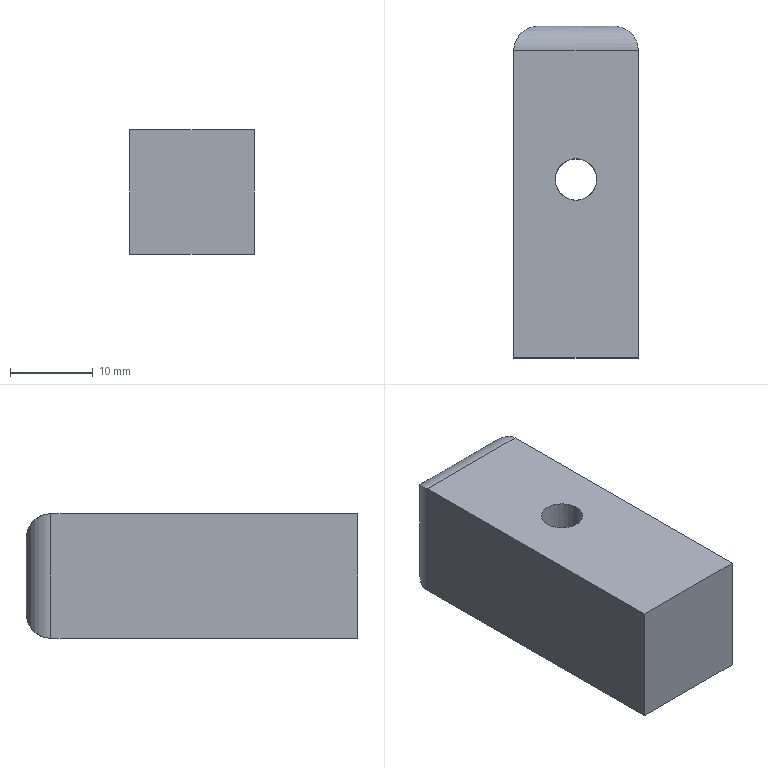Component | SolidWorks | SlideRailSupport-1 | 1 solid | 19 faces | box 15 x 40 x 15 mm | volume 8467 mm3 | cylinder 12 | plane 7 | commonest cylinder face diameters 5 x8 6 x4
build123d program:
from build123d import *

# Parameters (mm, degrees)
SKETCH1_W           = 15
SKETCH1_H           = 15
BOSS_EXTRUDE1_DEPTH = 20
FILLET1_R           = 3
SKETCH2_R           = 2.5
CUT_EXTRUDE1_DEPTH  = 25
SKETCH3_R           = 2.5
CUT_EXTRUDE2_DEPTH  = 11


with BuildPart() as part:
    # Sketch1 → Boss-Extrude1 (new, symmetric)
    with BuildSketch(Plane(origin=(0, 0, 0), x_dir=(0, 0, -1), z_dir=(1, 0, 0))):
        Rectangle(SKETCH1_W, SKETCH1_H)
    extrude(amount=BOSS_EXTRUDE1_DEPTH, both=True)

    # Fillet1
    fillet1_edges = [part.edges().sort_by_distance(p)[0] for p in [
        (-20, -7.5, 0),
        (-20, 0, 7.5),
        (-20, 7.5, 0),
        (-20, 0, -7.5),
    ]]
    fillet(fillet1_edges, radius=FILLET1_R)

    # Sketch2 → Cut-Extrude1 (cut, symmetric)
    with BuildSketch(Plane(origin=(0, 7.5, 0), x_dir=(1, 0, 0), z_dir=(0, 1, 0))):
        with Locations(Location((-1.5, 0, 0), (0, 0, 270))):
            Circle(SKETCH2_R)
    extrude(amount=CUT_EXTRUDE1_DEPTH, both=True, mode=Mode.SUBTRACT)

    # Sketch3 → Cut-Extrude2 (cut)
    with BuildSketch(Plane(origin=(0, 0, -7.5), x_dir=(-1, 0, 0), z_dir=(0, 0, -1))):
        with Locations(Location((1.5, 0, 0), (0, 0, 90))):
            Circle(SKETCH3_R)
    extrude(amount=-CUT_EXTRUDE2_DEPTH, mode=Mode.SUBTRACT)


solid = part.part

# Placed as in the assembly
solid = solid.moved(Location((-191.5, 218.5, 125), (90, -90, 0)))
STEP:
#1=CARTESIAN_POINT('',(-7.677,8.661,4.823));
#2=VERTEX_POINT('',#1);
#3=CARTESIAN_POINT('',(-7.677,8.661,5.02));
#4=VERTEX_POINT('',#3);
#5=CARTESIAN_POINT('',(-7.677,8.661,4.921));
#6=DIRECTION('',(1.,0.,0.));
#7=DIRECTION('',(0.,0.,1.));
#8=AXIS2_PLACEMENT_3D('',#5,#6,#7);
#9=CIRCLE('',#8,0.09843);
#10=EDGE_CURVE('',#2,#4,#9,.T.);
#11=ORIENTED_EDGE('',*,*,#10,.F.);
#12=CARTESIAN_POINT('',(-7.638,8.661,4.823));
#13=VERTEX_POINT('',#12);
#14=CARTESIAN_POINT('',(-7.677,8.661,4.823));
#15=DIRECTION('',(1.,0.,0.));
#16=VECTOR('',#15,39.37);
#17=LINE('',#14,#16);
#18=EDGE_CURVE('',#2,#13,#17,.T.);
#19=ORIENTED_EDGE('',*,*,#18,.T.);
#20=CARTESIAN_POINT('',(-7.539,8.76,4.921));
#21=VERTEX_POINT('',#20);
#22=CARTESIAN_POINT('',(-7.539,8.76,4.921));
#23=CARTESIAN_POINT('',(-7.597,8.76,4.864));
#24=CARTESIAN_POINT('',(-7.638,8.719,4.823));
#25=CARTESIAN_POINT('',(-7.638,8.661,4.823));
#26=(BOUNDED_CURVE()B_SPLINE_CURVE(3,(#22,#23,#24,#25),.UNSPECIFIED.,.F.,.T.)B_SPLINE_CURVE_WITH_KNOTS((4,4),(1.571,3.142),.UNSPECIFIED.)CURVE()GEOMETRIC_REPRESENTATION_ITEM()RATIONAL_B_SPLINE_CURVE((1.,0.8047,0.8047,1.))REPRESENTATION_ITEM(''));
#27=EDGE_CURVE('',#21,#13,#26,.T.);
#28=ORIENTED_EDGE('',*,*,#27,.F.);
#29=CARTESIAN_POINT('',(-7.638,8.661,5.02));
#30=VERTEX_POINT('',#29);
#31=CARTESIAN_POINT('',(-7.638,8.661,5.02));
#32=CARTESIAN_POINT('',(-7.638,8.719,5.02));
#33=CARTESIAN_POINT('',(-7.597,8.76,4.979));
#34=CARTESIAN_POINT('',(-7.539,8.76,4.921));
#35=(BOUNDED_CURVE()B_SPLINE_CURVE(3,(#31,#32,#33,#34),.UNSPECIFIED.,.F.,.T.)B_SPLINE_CURVE_WITH_KNOTS((4,4),(0.,1.571),.UNSPECIFIED.)CURVE()GEOMETRIC_REPRESENTATION_ITEM()RATIONAL_B_SPLINE_CURVE((1.,0.8047,0.8047,1.))REPRESENTATION_ITEM(''));
#36=EDGE_CURVE('',#30,#21,#35,.T.);
#37=ORIENTED_EDGE('',*,*,#36,.F.);
#38=CARTESIAN_POINT('',(-7.677,8.661,5.02));
#39=DIRECTION('',(1.,0.,0.));
#40=VECTOR('',#39,39.37);
#41=LINE('',#38,#40);
#42=EDGE_CURVE('',#4,#30,#41,.T.);
#43=ORIENTED_EDGE('',*,*,#42,.F.);
#44=EDGE_LOOP('',(#11,#19,#28,#37,#43));
#45=FACE_OUTER_BOUND('',#44,.T.);
#46=CARTESIAN_POINT('',(-7.677,8.661,4.921));
#47=DIRECTION('',(1.,0.,0.));
#48=DIRECTION('',(0.,0.,1.));
#49=AXIS2_PLACEMENT_3D('',#46,#47,#48);
#50=CYLINDRICAL_SURFACE('',#49,0.09843);
#51=ADVANCED_FACE('',(#45),#50,.F.);
#52=CARTESIAN_POINT('',(-7.441,8.661,4.823));
#53=VERTEX_POINT('',#52);
#54=CARTESIAN_POINT('',(-7.441,8.661,4.823));
#55=CARTESIAN_POINT('',(-7.441,8.719,4.823));
#56=CARTESIAN_POINT('',(-7.482,8.76,4.864));
#57=CARTESIAN_POINT('',(-7.539,8.76,4.921));
#58=(BOUNDED_CURVE()B_SPLINE_CURVE(3,(#54,#55,#56,#57),.UNSPECIFIED.,.F.,.F.)B_SPLINE_CURVE_WITH_KNOTS((4,4),(3.142,4.712),.UNSPECIFIED.)CURVE()GEOMETRIC_REPRESENTATION_ITEM()RATIONAL_B_SPLINE_CURVE((1.,0.8047,0.8047,1.))REPRESENTATION_ITEM(''));
#59=EDGE_CURVE('',#53,#21,#58,.T.);
#60=ORIENTED_EDGE('',*,*,#59,.F.);
#61=CARTESIAN_POINT('',(-7.244,8.661,4.823));
#62=VERTEX_POINT('',#61);
#63=CARTESIAN_POINT('',(-7.677,8.661,4.823));
#64=DIRECTION('',(1.,0.,0.));
#65=VECTOR('',#64,39.37);
#66=LINE('',#63,#65);
#67=EDGE_CURVE('',#53,#62,#66,.T.);
#68=ORIENTED_EDGE('',*,*,#67,.T.);
#69=CARTESIAN_POINT('',(-7.244,8.661,5.02));
#70=VERTEX_POINT('',#69);
#71=CARTESIAN_POINT('',(-7.244,8.661,4.921));
#72=DIRECTION('',(1.,0.,0.));
#73=DIRECTION('',(0.,0.,1.));
#74=AXIS2_PLACEMENT_3D('',#71,#72,#73);
#75=CIRCLE('',#74,0.09843);
#76=EDGE_CURVE('',#62,#70,#75,.T.);
#77=ORIENTED_EDGE('',*,*,#76,.T.);
#78=CARTESIAN_POINT('',(-7.441,8.661,5.02));
#79=VERTEX_POINT('',#78);
#80=CARTESIAN_POINT('',(-7.677,8.661,5.02));
#81=DIRECTION('',(1.,0.,0.));
#82=VECTOR('',#81,39.37);
#83=LINE('',#80,#82);
#84=EDGE_CURVE('',#79,#70,#83,.T.);
#85=ORIENTED_EDGE('',*,*,#84,.F.);
#86=CARTESIAN_POINT('',(-7.539,8.76,4.921));
#87=CARTESIAN_POINT('',(-7.482,8.76,4.979));
#88=CARTESIAN_POINT('',(-7.441,8.719,5.02));
#89=CARTESIAN_POINT('',(-7.441,8.661,5.02));
#90=(BOUNDED_CURVE()B_SPLINE_CURVE(3,(#86,#87,#88,#89),.UNSPECIFIED.,.F.,.F.)B_SPLINE_CURVE_WITH_KNOTS((4,4),(4.712,6.283),.UNSPECIFIED.)CURVE()GEOMETRIC_REPRESENTATION_ITEM()RATIONAL_B_SPLINE_CURVE((1.,0.8047,0.8047,1.))REPRESENTATION_ITEM(''));
#91=EDGE_CURVE('',#21,#79,#90,.T.);
#92=ORIENTED_EDGE('',*,*,#91,.F.);
#93=EDGE_LOOP('',(#60,#68,#77,#85,#92));
#94=FACE_OUTER_BOUND('',#93,.T.);
#95=CARTESIAN_POINT('',(-7.677,8.661,4.921));
#96=DIRECTION('',(1.,0.,0.));
#97=DIRECTION('',(0.,0.,1.));
#98=AXIS2_PLACEMENT_3D('',#95,#96,#97);
#99=CYLINDRICAL_SURFACE('',#98,0.09843);
#100=ADVANCED_FACE('',(#94),#99,.F.);
#101=CARTESIAN_POINT('',(-7.441,8.661,4.626));
#102=VERTEX_POINT('',#101);
#103=CARTESIAN_POINT('',(-7.638,8.661,4.626));
#104=VERTEX_POINT('',#103);
#105=CARTESIAN_POINT('',(-7.539,8.661,4.626));
#106=DIRECTION('',(0.,0.,1.));
#107=DIRECTION('',(-1.,0.,0.));
#108=AXIS2_PLACEMENT_3D('',#105,#106,#107);
#109=CIRCLE('',#108,0.09843);
#110=EDGE_CURVE('',#102,#104,#109,.T.);
#111=ORIENTED_EDGE('',*,*,#110,.F.);
#112=CARTESIAN_POINT('',(-7.441,8.661,4.232));
#113=DIRECTION('',(-0.,0.,1.));
#114=VECTOR('',#113,39.37);
#115=LINE('',#112,#114);
#116=EDGE_CURVE('',#102,#53,#115,.T.);
#117=ORIENTED_EDGE('',*,*,#116,.T.);
#118=ORIENTED_EDGE('',*,*,#59,.T.);
#119=ORIENTED_EDGE('',*,*,#27,.T.);
#120=CARTESIAN_POINT('',(-7.638,8.661,4.232));
#121=DIRECTION('',(-0.,0.,1.));
#122=VECTOR('',#121,39.37);
#123=LINE('',#120,#122);
#124=EDGE_CURVE('',#104,#13,#123,.T.);
#125=ORIENTED_EDGE('',*,*,#124,.F.);
#126=EDGE_LOOP('',(#111,#117,#118,#119,#125));
#127=FACE_OUTER_BOUND('',#126,.T.);
#128=CARTESIAN_POINT('',(-7.539,8.661,4.232));
#129=DIRECTION('',(-0.,0.,1.));
#130=DIRECTION('',(-1.,0.,0.));
#131=AXIS2_PLACEMENT_3D('',#128,#129,#130);
#132=CYLINDRICAL_SURFACE('',#131,0.09843);
#133=ADVANCED_FACE('',(#127),#132,.F.);
#134=ORIENTED_EDGE('',*,*,#91,.T.);
#135=CARTESIAN_POINT('',(-7.441,8.661,5.217));
#136=VERTEX_POINT('',#135);
#137=CARTESIAN_POINT('',(-7.441,8.661,4.232));
#138=DIRECTION('',(-0.,0.,1.));
#139=VECTOR('',#138,39.37);
#140=LINE('',#137,#139);
#141=EDGE_CURVE('',#79,#136,#140,.T.);
#142=ORIENTED_EDGE('',*,*,#141,.T.);
#143=CARTESIAN_POINT('',(-7.638,8.661,5.217));
#144=VERTEX_POINT('',#143);
#145=CARTESIAN_POINT('',(-7.539,8.661,5.217));
#146=DIRECTION('',(0.,-0.,-1.));
#147=DIRECTION('',(1.,0.,0.));
#148=AXIS2_PLACEMENT_3D('',#145,#146,#147);
#149=CIRCLE('',#148,0.09843);
#150=EDGE_CURVE('',#144,#136,#149,.T.);
#151=ORIENTED_EDGE('',*,*,#150,.F.);
#152=CARTESIAN_POINT('',(-7.638,8.661,4.232));
#153=DIRECTION('',(-0.,0.,1.));
#154=VECTOR('',#153,39.37);
#155=LINE('',#152,#154);
#156=EDGE_CURVE('',#30,#144,#155,.T.);
#157=ORIENTED_EDGE('',*,*,#156,.F.);
#158=ORIENTED_EDGE('',*,*,#36,.T.);
#159=EDGE_LOOP('',(#134,#142,#151,#157,#158));
#160=FACE_OUTER_BOUND('',#159,.T.);
#161=CARTESIAN_POINT('',(-7.539,8.661,4.232));
#162=DIRECTION('',(-0.,0.,1.));
#163=DIRECTION('',(-1.,0.,0.));
#164=AXIS2_PLACEMENT_3D('',#161,#162,#163);
#165=CYLINDRICAL_SURFACE('',#164,0.09843);
#166=ADVANCED_FACE('',(#160),#165,.F.);
#167=ORIENTED_EDGE('',*,*,#141,.F.);
#168=CARTESIAN_POINT('',(-7.539,8.563,4.921));
#169=VERTEX_POINT('',#168);
#170=CARTESIAN_POINT('',(-7.441,8.661,5.02));
#171=CARTESIAN_POINT('',(-7.441,8.604,5.02));
#172=CARTESIAN_POINT('',(-7.482,8.563,4.979));
#173=CARTESIAN_POINT('',(-7.539,8.563,4.921));
#174=(BOUNDED_CURVE()B_SPLINE_CURVE(3,(#170,#171,#172,#173),.UNSPECIFIED.,.F.,.F.)B_SPLINE_CURVE_WITH_KNOTS((4,4),(0.,1.571),.UNSPECIFIED.)CURVE()GEOMETRIC_REPRESENTATION_ITEM()RATIONAL_B_SPLINE_CURVE((1.,0.8047,0.8047,1.))REPRESENTATION_ITEM(''));
#175=EDGE_CURVE('',#79,#169,#174,.T.);
#176=ORIENTED_EDGE('',*,*,#175,.T.);
#177=CARTESIAN_POINT('',(-7.539,8.563,4.921));
#178=CARTESIAN_POINT('',(-7.597,8.563,4.979));
#179=CARTESIAN_POINT('',(-7.638,8.604,5.02));
#180=CARTESIAN_POINT('',(-7.638,8.661,5.02));
#181=(BOUNDED_CURVE()B_SPLINE_CURVE(3,(#177,#178,#179,#180),.UNSPECIFIED.,.F.,.T.)B_SPLINE_CURVE_WITH_KNOTS((4,4),(4.712,6.283),.UNSPECIFIED.)CURVE()GEOMETRIC_REPRESENTATION_ITEM()RATIONAL_B_SPLINE_CURVE((1.,0.8047,0.8047,1.))REPRESENTATION_ITEM(''));
#182=EDGE_CURVE('',#169,#30,#181,.T.);
#183=ORIENTED_EDGE('',*,*,#182,.T.);
#184=ORIENTED_EDGE('',*,*,#156,.T.);
#185=CARTESIAN_POINT('',(-7.539,8.661,5.217));
#186=DIRECTION('',(0.,-0.,-1.));
#187=DIRECTION('',(1.,0.,0.));
#188=AXIS2_PLACEMENT_3D('',#185,#186,#187);
#189=CIRCLE('',#188,0.09843);
#190=EDGE_CURVE('',#136,#144,#189,.T.);
#191=ORIENTED_EDGE('',*,*,#190,.F.);
#192=EDGE_LOOP('',(#167,#176,#183,#184,#191));
#193=FACE_OUTER_BOUND('',#192,.T.);
#194=CARTESIAN_POINT('',(-7.539,8.661,4.232));
#195=DIRECTION('',(-0.,0.,1.));
#196=DIRECTION('',(-1.,0.,0.));
#197=AXIS2_PLACEMENT_3D('',#194,#195,#196);
#198=CYLINDRICAL_SURFACE('',#197,0.09843);
#199=ADVANCED_FACE('',(#193),#198,.F.);
#200=CARTESIAN_POINT('',(-7.244,8.661,4.921));
#201=DIRECTION('',(1.,0.,0.));
#202=DIRECTION('',(0.,0.,1.));
#203=AXIS2_PLACEMENT_3D('',#200,#201,#202);
#204=CIRCLE('',#203,0.09843);
#205=EDGE_CURVE('',#70,#62,#204,.T.);
#206=ORIENTED_EDGE('',*,*,#205,.F.);
#207=ORIENTED_EDGE('',*,*,#76,.F.);
#208=EDGE_LOOP('',(#206,#207));
#209=FACE_BOUND('',#208,.T.);
#210=CARTESIAN_POINT('',(-7.244,7.815,4.626));
#211=VERTEX_POINT('',#210);
#212=CARTESIAN_POINT('',(-7.244,9.272,4.626));
#213=VERTEX_POINT('',#212);
#214=CARTESIAN_POINT('',(-7.244,7.815,4.626));
#215=DIRECTION('',(-0.,1.,-0.));
#216=VECTOR('',#215,39.37);
#217=LINE('',#214,#216);
#218=EDGE_CURVE('',#211,#213,#217,.T.);
#219=ORIENTED_EDGE('',*,*,#218,.T.);
#220=CARTESIAN_POINT('',(-7.244,9.272,5.217));
#221=VERTEX_POINT('',#220);
#222=CARTESIAN_POINT('',(-7.244,9.272,5.217));
#223=DIRECTION('',(-0.,0.,1.));
#224=VECTOR('',#223,39.37);
#225=LINE('',#222,#224);
#226=EDGE_CURVE('',#213,#221,#225,.T.);
#227=ORIENTED_EDGE('',*,*,#226,.T.);
#228=CARTESIAN_POINT('',(-7.244,7.815,5.217));
#229=VERTEX_POINT('',#228);
#230=CARTESIAN_POINT('',(-7.244,7.815,5.217));
#231=DIRECTION('',(-0.,1.,-0.));
#232=VECTOR('',#231,39.37);
#233=LINE('',#230,#232);
#234=EDGE_CURVE('',#229,#221,#233,.T.);
#235=ORIENTED_EDGE('',*,*,#234,.F.);
#236=CARTESIAN_POINT('',(-7.244,7.815,5.217));
#237=DIRECTION('',(-0.,0.,1.));
#238=VECTOR('',#237,39.37);
#239=LINE('',#236,#238);
#240=EDGE_CURVE('',#211,#229,#239,.T.);
#241=ORIENTED_EDGE('',*,*,#240,.F.);
#242=EDGE_LOOP('',(#219,#227,#235,#241));
#243=FACE_OUTER_BOUND('',#242,.T.);
#244=CARTESIAN_POINT('',(-7.244,7.815,5.217));
#245=DIRECTION('',(-1.,-0.,-0.));
#246=DIRECTION('',(0.,-0.,-1.));
#247=AXIS2_PLACEMENT_3D('',#244,#245,#246);
#248=PLANE('',#247);
#249=ADVANCED_FACE('',(#209,#243),#248,.F.);
#250=ORIENTED_EDGE('',*,*,#150,.T.);
#251=ORIENTED_EDGE('',*,*,#190,.T.);
#252=EDGE_LOOP('',(#250,#251));
#253=FACE_BOUND('',#252,.T.);
#254=ORIENTED_EDGE('',*,*,#234,.T.);
#255=CARTESIAN_POINT('',(-7.835,9.272,5.217));
#256=VERTEX_POINT('',#255);
#257=CARTESIAN_POINT('',(-7.835,9.272,5.217));
#258=DIRECTION('',(-1.,-0.,0.));
#259=VECTOR('',#258,39.37);
#260=LINE('',#257,#259);
#261=EDGE_CURVE('',#221,#256,#260,.T.);
#262=ORIENTED_EDGE('',*,*,#261,.T.);
#263=CARTESIAN_POINT('',(-7.835,7.815,5.217));
#264=VERTEX_POINT('',#263);
#265=CARTESIAN_POINT('',(-7.835,7.815,5.217));
#266=DIRECTION('',(-0.,1.,-0.));
#267=VECTOR('',#266,39.37);
#268=LINE('',#265,#267);
#269=EDGE_CURVE('',#264,#256,#268,.T.);
#270=ORIENTED_EDGE('',*,*,#269,.F.);
#271=CARTESIAN_POINT('',(-7.835,7.815,5.217));
#272=DIRECTION('',(-1.,-0.,0.));
#273=VECTOR('',#272,39.37);
#274=LINE('',#271,#273);
#275=EDGE_CURVE('',#229,#264,#274,.T.);
#276=ORIENTED_EDGE('',*,*,#275,.F.);
#277=EDGE_LOOP('',(#254,#262,#270,#276));
#278=FACE_OUTER_BOUND('',#277,.T.);
#279=CARTESIAN_POINT('',(-7.835,7.815,5.217));
#280=DIRECTION('',(0.,-0.,-1.));
#281=DIRECTION('',(1.,0.,-0.));
#282=AXIS2_PLACEMENT_3D('',#279,#280,#281);
#283=PLANE('',#282);
#284=ADVANCED_FACE('',(#253,#278),#283,.F.);
#285=ORIENTED_EDGE('',*,*,#269,.T.);
#286=CARTESIAN_POINT('',(-7.835,9.272,4.626));
#287=VERTEX_POINT('',#286);
#288=CARTESIAN_POINT('',(-7.835,9.272,5.217));
#289=DIRECTION('',(0.,-0.,-1.));
#290=VECTOR('',#289,39.37);
#291=LINE('',#288,#290);
#292=EDGE_CURVE('',#256,#287,#291,.T.);
#293=ORIENTED_EDGE('',*,*,#292,.T.);
#294=CARTESIAN_POINT('',(-7.835,7.815,4.626));
#295=VERTEX_POINT('',#294);
#296=CARTESIAN_POINT('',(-7.835,7.815,4.626));
#297=DIRECTION('',(-0.,1.,-0.));
#298=VECTOR('',#297,39.37);
#299=LINE('',#296,#298);
#300=EDGE_CURVE('',#295,#287,#299,.T.);
#301=ORIENTED_EDGE('',*,*,#300,.F.);
#302=CARTESIAN_POINT('',(-7.835,7.815,5.217));
#303=DIRECTION('',(0.,-0.,-1.));
#304=VECTOR('',#303,39.37);
#305=LINE('',#302,#304);
#306=EDGE_CURVE('',#264,#295,#305,.T.);
#307=ORIENTED_EDGE('',*,*,#306,.F.);
#308=EDGE_LOOP('',(#285,#293,#301,#307));
#309=FACE_OUTER_BOUND('',#308,.T.);
#310=CARTESIAN_POINT('',(-7.835,7.815,5.217));
#311=DIRECTION('',(1.,0.,0.));
#312=DIRECTION('',(-0.,0.,1.));
#313=AXIS2_PLACEMENT_3D('',#310,#311,#312);
#314=PLANE('',#313);
#315=ADVANCED_FACE('',(#309),#314,.F.);
#316=CARTESIAN_POINT('',(-7.539,8.661,4.626));
#317=DIRECTION('',(0.,0.,1.));
#318=DIRECTION('',(-1.,0.,0.));
#319=AXIS2_PLACEMENT_3D('',#316,#317,#318);
#320=CIRCLE('',#319,0.09843);
#321=EDGE_CURVE('',#104,#102,#320,.T.);
#322=ORIENTED_EDGE('',*,*,#321,.T.);
#323=ORIENTED_EDGE('',*,*,#110,.T.);
#324=EDGE_LOOP('',(#322,#323));
#325=FACE_BOUND('',#324,.T.);
#326=ORIENTED_EDGE('',*,*,#300,.T.);
#327=CARTESIAN_POINT('',(-7.835,9.272,4.626));
#328=DIRECTION('',(1.,0.,-0.));
#329=VECTOR('',#328,39.37);
#330=LINE('',#327,#329);
#331=EDGE_CURVE('',#287,#213,#330,.T.);
#332=ORIENTED_EDGE('',*,*,#331,.T.);
#333=ORIENTED_EDGE('',*,*,#218,.F.);
#334=CARTESIAN_POINT('',(-7.835,7.815,4.626));
#335=DIRECTION('',(1.,0.,-0.));
#336=VECTOR('',#335,39.37);
#337=LINE('',#334,#336);
#338=EDGE_CURVE('',#295,#211,#337,.T.);
#339=ORIENTED_EDGE('',*,*,#338,.F.);
#340=EDGE_LOOP('',(#326,#332,#333,#339));
#341=FACE_OUTER_BOUND('',#340,.T.);
#342=CARTESIAN_POINT('',(-7.835,7.815,4.626));
#343=DIRECTION('',(0.,0.,1.));
#344=DIRECTION('',(-1.,-0.,0.));
#345=AXIS2_PLACEMENT_3D('',#342,#343,#344);
#346=PLANE('',#345);
#347=ADVANCED_FACE('',(#325,#341),#346,.F.);
#348=ORIENTED_EDGE('',*,*,#240,.T.);
#349=ORIENTED_EDGE('',*,*,#275,.T.);
#350=ORIENTED_EDGE('',*,*,#306,.T.);
#351=ORIENTED_EDGE('',*,*,#338,.T.);
#352=EDGE_LOOP('',(#348,#349,#350,#351));
#353=FACE_OUTER_BOUND('',#352,.T.);
#354=CARTESIAN_POINT('',(-7.539,7.815,4.921));
#355=DIRECTION('',(0.,-1.,0.));
#356=DIRECTION('',(1.,0.,-0.));
#357=AXIS2_PLACEMENT_3D('',#354,#355,#356);
#358=PLANE('',#357);
#359=ADVANCED_FACE('',(#353),#358,.T.);
#360=CARTESIAN_POINT('',(-7.717,9.39,4.744));
#361=VERTEX_POINT('',#360);
#362=CARTESIAN_POINT('',(-7.717,9.39,5.098));
#363=VERTEX_POINT('',#362);
#364=CARTESIAN_POINT('',(-7.717,9.39,4.921));
#365=DIRECTION('',(-0.,0.,1.));
#366=VECTOR('',#365,39.37);
#367=LINE('',#364,#366);
#368=EDGE_CURVE('',#361,#363,#367,.T.);
#369=ORIENTED_EDGE('',*,*,#368,.T.);
#370=CARTESIAN_POINT('',(-7.362,9.39,5.098));
#371=VERTEX_POINT('',#370);
#372=CARTESIAN_POINT('',(-7.539,9.39,5.098));
#373=DIRECTION('',(1.,0.,-0.));
#374=VECTOR('',#373,39.37);
#375=LINE('',#372,#374);
#376=EDGE_CURVE('',#363,#371,#375,.T.);
#377=ORIENTED_EDGE('',*,*,#376,.T.);
#378=CARTESIAN_POINT('',(-7.362,9.39,4.744));
#379=VERTEX_POINT('',#378);
#380=CARTESIAN_POINT('',(-7.362,9.39,4.921));
#381=DIRECTION('',(0.,-0.,-1.));
#382=VECTOR('',#381,39.37);
#383=LINE('',#380,#382);
#384=EDGE_CURVE('',#371,#379,#383,.T.);
#385=ORIENTED_EDGE('',*,*,#384,.T.);
#386=CARTESIAN_POINT('',(-7.539,9.39,4.744));
#387=DIRECTION('',(-1.,-0.,0.));
#388=VECTOR('',#387,39.37);
#389=LINE('',#386,#388);
#390=EDGE_CURVE('',#379,#361,#389,.T.);
#391=ORIENTED_EDGE('',*,*,#390,.T.);
#392=EDGE_LOOP('',(#369,#377,#385,#391));
#393=FACE_OUTER_BOUND('',#392,.T.);
#394=CARTESIAN_POINT('',(-7.539,9.39,4.921));
#395=DIRECTION('',(0.,-1.,0.));
#396=DIRECTION('',(1.,0.,-0.));
#397=AXIS2_PLACEMENT_3D('',#394,#395,#396);
#398=PLANE('',#397);
#399=ADVANCED_FACE('',(#393),#398,.F.);
#400=CARTESIAN_POINT('',(-7.717,9.39,4.744));
#401=CARTESIAN_POINT('',(-7.786,9.39,4.675));
#402=CARTESIAN_POINT('',(-7.835,9.341,4.626));
#403=CARTESIAN_POINT('',(-7.835,9.272,4.626));
#404=(BOUNDED_CURVE()B_SPLINE_CURVE(3,(#400,#401,#402,#403),.UNSPECIFIED.,.F.,.F.)B_SPLINE_CURVE_WITH_KNOTS((4,4),(1.571,3.142),.UNSPECIFIED.)CURVE()GEOMETRIC_REPRESENTATION_ITEM()RATIONAL_B_SPLINE_CURVE((1.,0.8047,0.8047,1.))REPRESENTATION_ITEM(''));
#405=EDGE_CURVE('',#361,#287,#404,.T.);
#406=ORIENTED_EDGE('',*,*,#405,.F.);
#407=ORIENTED_EDGE('',*,*,#390,.F.);
#408=CARTESIAN_POINT('',(-7.244,9.272,4.626));
#409=CARTESIAN_POINT('',(-7.244,9.341,4.626));
#410=CARTESIAN_POINT('',(-7.293,9.39,4.675));
#411=CARTESIAN_POINT('',(-7.362,9.39,4.744));
#412=(BOUNDED_CURVE()B_SPLINE_CURVE(3,(#408,#409,#410,#411),.UNSPECIFIED.,.F.,.F.)B_SPLINE_CURVE_WITH_KNOTS((4,4),(3.142,4.712),.UNSPECIFIED.)CURVE()GEOMETRIC_REPRESENTATION_ITEM()RATIONAL_B_SPLINE_CURVE((1.,0.8047,0.8047,1.))REPRESENTATION_ITEM(''));
#413=EDGE_CURVE('',#213,#379,#412,.T.);
#414=ORIENTED_EDGE('',*,*,#413,.F.);
#415=ORIENTED_EDGE('',*,*,#331,.F.);
#416=EDGE_LOOP('',(#406,#407,#414,#415));
#417=FACE_OUTER_BOUND('',#416,.T.);
#418=CARTESIAN_POINT('',(-7.835,9.272,4.744));
#419=DIRECTION('',(1.,0.,-0.));
#420=DIRECTION('',(0.,1.,0.));
#421=AXIS2_PLACEMENT_3D('',#418,#419,#420);
#422=CYLINDRICAL_SURFACE('',#421,0.1181);
#423=ADVANCED_FACE('',(#417),#422,.T.);
#424=ORIENTED_EDGE('',*,*,#413,.T.);
#425=ORIENTED_EDGE('',*,*,#384,.F.);
#426=CARTESIAN_POINT('',(-7.244,9.272,5.217));
#427=CARTESIAN_POINT('',(-7.244,9.341,5.217));
#428=CARTESIAN_POINT('',(-7.293,9.39,5.168));
#429=CARTESIAN_POINT('',(-7.362,9.39,5.098));
#430=(BOUNDED_CURVE()B_SPLINE_CURVE(3,(#426,#427,#428,#429),.UNSPECIFIED.,.F.,.F.)B_SPLINE_CURVE_WITH_KNOTS((4,4),(0.,1.571),.UNSPECIFIED.)CURVE()GEOMETRIC_REPRESENTATION_ITEM()RATIONAL_B_SPLINE_CURVE((1.,0.8047,0.8047,1.))REPRESENTATION_ITEM(''));
#431=EDGE_CURVE('',#221,#371,#430,.T.);
#432=ORIENTED_EDGE('',*,*,#431,.F.);
#433=ORIENTED_EDGE('',*,*,#226,.F.);
#434=EDGE_LOOP('',(#424,#425,#432,#433));
#435=FACE_OUTER_BOUND('',#434,.T.);
#436=CARTESIAN_POINT('',(-7.362,9.272,5.217));
#437=DIRECTION('',(-0.,0.,1.));
#438=DIRECTION('',(-1.,0.,0.));
#439=AXIS2_PLACEMENT_3D('',#436,#437,#438);
#440=CYLINDRICAL_SURFACE('',#439,0.1181);
#441=ADVANCED_FACE('',(#435),#440,.T.);
#442=ORIENTED_EDGE('',*,*,#405,.T.);
#443=ORIENTED_EDGE('',*,*,#292,.F.);
#444=CARTESIAN_POINT('',(-7.717,9.39,5.098));
#445=CARTESIAN_POINT('',(-7.786,9.39,5.168));
#446=CARTESIAN_POINT('',(-7.835,9.341,5.217));
#447=CARTESIAN_POINT('',(-7.835,9.272,5.217));
#448=(BOUNDED_CURVE()B_SPLINE_CURVE(3,(#444,#445,#446,#447),.UNSPECIFIED.,.F.,.F.)B_SPLINE_CURVE_WITH_KNOTS((4,4),(1.571,3.142),.UNSPECIFIED.)CURVE()GEOMETRIC_REPRESENTATION_ITEM()RATIONAL_B_SPLINE_CURVE((1.,0.8047,0.8047,1.))REPRESENTATION_ITEM(''));
#449=EDGE_CURVE('',#363,#256,#448,.T.);
#450=ORIENTED_EDGE('',*,*,#449,.F.);
#451=ORIENTED_EDGE('',*,*,#368,.F.);
#452=EDGE_LOOP('',(#442,#443,#450,#451));
#453=FACE_OUTER_BOUND('',#452,.T.);
#454=CARTESIAN_POINT('',(-7.717,9.272,5.217));
#455=DIRECTION('',(0.,-0.,-1.));
#456=DIRECTION('',(1.,0.,0.));
#457=AXIS2_PLACEMENT_3D('',#454,#455,#456);
#458=CYLINDRICAL_SURFACE('',#457,0.1181);
#459=ADVANCED_FACE('',(#453),#458,.T.);
#460=ORIENTED_EDGE('',*,*,#431,.T.);
#461=ORIENTED_EDGE('',*,*,#376,.F.);
#462=ORIENTED_EDGE('',*,*,#449,.T.);
#463=ORIENTED_EDGE('',*,*,#261,.F.);
#464=EDGE_LOOP('',(#460,#461,#462,#463));
#465=FACE_OUTER_BOUND('',#464,.T.);
#466=CARTESIAN_POINT('',(-7.835,9.272,5.098));
#467=DIRECTION('',(-1.,-0.,0.));
#468=DIRECTION('',(0.,0.,-1.));
#469=AXIS2_PLACEMENT_3D('',#466,#467,#468);
#470=CYLINDRICAL_SURFACE('',#469,0.1181);
#471=ADVANCED_FACE('',(#465),#470,.T.);
#472=ORIENTED_EDGE('',*,*,#116,.F.);
#473=ORIENTED_EDGE('',*,*,#321,.F.);
#474=ORIENTED_EDGE('',*,*,#124,.T.);
#475=CARTESIAN_POINT('',(-7.638,8.661,4.823));
#476=CARTESIAN_POINT('',(-7.638,8.604,4.823));
#477=CARTESIAN_POINT('',(-7.597,8.563,4.864));
#478=CARTESIAN_POINT('',(-7.539,8.563,4.921));
#479=(BOUNDED_CURVE()B_SPLINE_CURVE(3,(#475,#476,#477,#478),.UNSPECIFIED.,.F.,.F.)B_SPLINE_CURVE_WITH_KNOTS((4,4),(3.142,4.712),.UNSPECIFIED.)CURVE()GEOMETRIC_REPRESENTATION_ITEM()RATIONAL_B_SPLINE_CURVE((1.,0.8047,0.8047,1.))REPRESENTATION_ITEM(''));
#480=EDGE_CURVE('',#13,#169,#479,.T.);
#481=ORIENTED_EDGE('',*,*,#480,.T.);
#482=CARTESIAN_POINT('',(-7.539,8.563,4.921));
#483=CARTESIAN_POINT('',(-7.482,8.563,4.864));
#484=CARTESIAN_POINT('',(-7.441,8.604,4.823));
#485=CARTESIAN_POINT('',(-7.441,8.661,4.823));
#486=(BOUNDED_CURVE()B_SPLINE_CURVE(3,(#482,#483,#484,#485),.UNSPECIFIED.,.F.,.F.)B_SPLINE_CURVE_WITH_KNOTS((4,4),(1.571,3.142),.UNSPECIFIED.)CURVE()GEOMETRIC_REPRESENTATION_ITEM()RATIONAL_B_SPLINE_CURVE((1.,0.8047,0.8047,1.))REPRESENTATION_ITEM(''));
#487=EDGE_CURVE('',#169,#53,#486,.T.);
#488=ORIENTED_EDGE('',*,*,#487,.T.);
#489=EDGE_LOOP('',(#472,#473,#474,#481,#488));
#490=FACE_OUTER_BOUND('',#489,.T.);
#491=CARTESIAN_POINT('',(-7.539,8.661,4.232));
#492=DIRECTION('',(-0.,0.,1.));
#493=DIRECTION('',(-1.,0.,0.));
#494=AXIS2_PLACEMENT_3D('',#491,#492,#493);
#495=CYLINDRICAL_SURFACE('',#494,0.09843);
#496=ADVANCED_FACE('',(#490),#495,.F.);
#497=ORIENTED_EDGE('',*,*,#67,.F.);
#498=ORIENTED_EDGE('',*,*,#487,.F.);
#499=ORIENTED_EDGE('',*,*,#175,.F.);
#500=ORIENTED_EDGE('',*,*,#84,.T.);
#501=ORIENTED_EDGE('',*,*,#205,.T.);
#502=EDGE_LOOP('',(#497,#498,#499,#500,#501));
#503=FACE_OUTER_BOUND('',#502,.T.);
#504=CARTESIAN_POINT('',(-7.677,8.661,4.921));
#505=DIRECTION('',(1.,0.,0.));
#506=DIRECTION('',(0.,0.,1.));
#507=AXIS2_PLACEMENT_3D('',#504,#505,#506);
#508=CYLINDRICAL_SURFACE('',#507,0.09843);
#509=ADVANCED_FACE('',(#503),#508,.F.);
#510=ORIENTED_EDGE('',*,*,#18,.F.);
#511=CARTESIAN_POINT('',(-7.677,8.661,4.921));
#512=DIRECTION('',(1.,0.,0.));
#513=DIRECTION('',(0.,0.,1.));
#514=AXIS2_PLACEMENT_3D('',#511,#512,#513);
#515=CIRCLE('',#514,0.09843);
#516=EDGE_CURVE('',#4,#2,#515,.T.);
#517=ORIENTED_EDGE('',*,*,#516,.F.);
#518=ORIENTED_EDGE('',*,*,#42,.T.);
#519=ORIENTED_EDGE('',*,*,#182,.F.);
#520=ORIENTED_EDGE('',*,*,#480,.F.);
#521=EDGE_LOOP('',(#510,#517,#518,#519,#520));
#522=FACE_OUTER_BOUND('',#521,.T.);
#523=CARTESIAN_POINT('',(-7.677,8.661,4.921));
#524=DIRECTION('',(1.,0.,0.));
#525=DIRECTION('',(0.,0.,1.));
#526=AXIS2_PLACEMENT_3D('',#523,#524,#525);
#527=CYLINDRICAL_SURFACE('',#526,0.09843);
#528=ADVANCED_FACE('',(#522),#527,.F.);
#529=ORIENTED_EDGE('',*,*,#516,.T.);
#530=ORIENTED_EDGE('',*,*,#10,.T.);
#531=EDGE_LOOP('',(#529,#530));
#532=FACE_OUTER_BOUND('',#531,.T.);
#533=CARTESIAN_POINT('',(-7.677,8.661,4.921));
#534=DIRECTION('',(1.,0.,0.));
#535=DIRECTION('',(-0.,0.,1.));
#536=AXIS2_PLACEMENT_3D('',#533,#534,#535);
#537=PLANE('',#536);
#538=ADVANCED_FACE('',(#532),#537,.T.);
#539=CLOSED_SHELL('',(#51,#100,#133,#166,#199,#249,#284,#315,#347,#359,#399,#423,#441,#459,#471,#496,#509,#528,#538));
#540=MANIFOLD_SOLID_BREP('',#539);
#541=CARTESIAN_POINT('',(0.,0.,0.));
#542=DIRECTION('',(0.,0.,1.));
#543=DIRECTION('',(1.,0.,0.));
#544=AXIS2_PLACEMENT_3D('',#541,#542,#543);
#545=(LENGTH_UNIT()NAMED_UNIT(*)SI_UNIT($,.METRE.));
#546=LENGTH_MEASURE_WITH_UNIT(LENGTH_MEASURE(0.0254),#545);
#547=DIMENSIONAL_EXPONENTS(1.,0.,0.,0.,0.,0.,0.);
#548=(CONVERSION_BASED_UNIT('',#546)LENGTH_UNIT()NAMED_UNIT(#547));
#549=UNCERTAINTY_MEASURE_WITH_UNIT(LENGTH_MEASURE(0.00001),#548,'','');
#550=(NAMED_UNIT(*)PLANE_ANGLE_UNIT()SI_UNIT($,.RADIAN.));
#551=(NAMED_UNIT(*)SI_UNIT($,.STERADIAN.)SOLID_ANGLE_UNIT());
#552=(GEOMETRIC_REPRESENTATION_CONTEXT(3)GLOBAL_UNCERTAINTY_ASSIGNED_CONTEXT((#549))GLOBAL_UNIT_ASSIGNED_CONTEXT((#548,#550,#551))REPRESENTATION_CONTEXT('',''));
#553=ADVANCED_BREP_SHAPE_REPRESENTATION('',(#540,#544),#552);
#554=COLOUR_RGB('',0.7922,0.8196,0.9333);
#555=FILL_AREA_STYLE_COLOUR('',#554);
#556=FILL_AREA_STYLE('',(#555));
#557=SURFACE_STYLE_FILL_AREA(#556);
#558=SURFACE_SIDE_STYLE('',(#557));
#559=SURFACE_STYLE_USAGE(.BOTH.,#558);
#560=PRESENTATION_STYLE_ASSIGNMENT((#559));
#561=STYLED_ITEM('',(#560),#540);
#562=(LENGTH_UNIT()NAMED_UNIT(*)SI_UNIT($,.METRE.));
#563=LENGTH_MEASURE_WITH_UNIT(LENGTH_MEASURE(0.0254),#562);
#564=DIMENSIONAL_EXPONENTS(1.,0.,0.,0.,0.,0.,0.);
#565=(CONVERSION_BASED_UNIT('',#563)LENGTH_UNIT()NAMED_UNIT(#564));
#566=UNCERTAINTY_MEASURE_WITH_UNIT(LENGTH_MEASURE(0.00001),#565,'','');
#567=(NAMED_UNIT(*)PLANE_ANGLE_UNIT()SI_UNIT($,.RADIAN.));
#568=(NAMED_UNIT(*)SI_UNIT($,.STERADIAN.)SOLID_ANGLE_UNIT());
#569=(GEOMETRIC_REPRESENTATION_CONTEXT(3)GLOBAL_UNCERTAINTY_ASSIGNED_CONTEXT((#566))GLOBAL_UNIT_ASSIGNED_CONTEXT((#565,#567,#568))REPRESENTATION_CONTEXT('',''));
#570=MECHANICAL_DESIGN_GEOMETRIC_PRESENTATION_REPRESENTATION('',(#561),#569);
#571=PRESENTATION_LAYER_ASSIGNMENT('','',(#561));